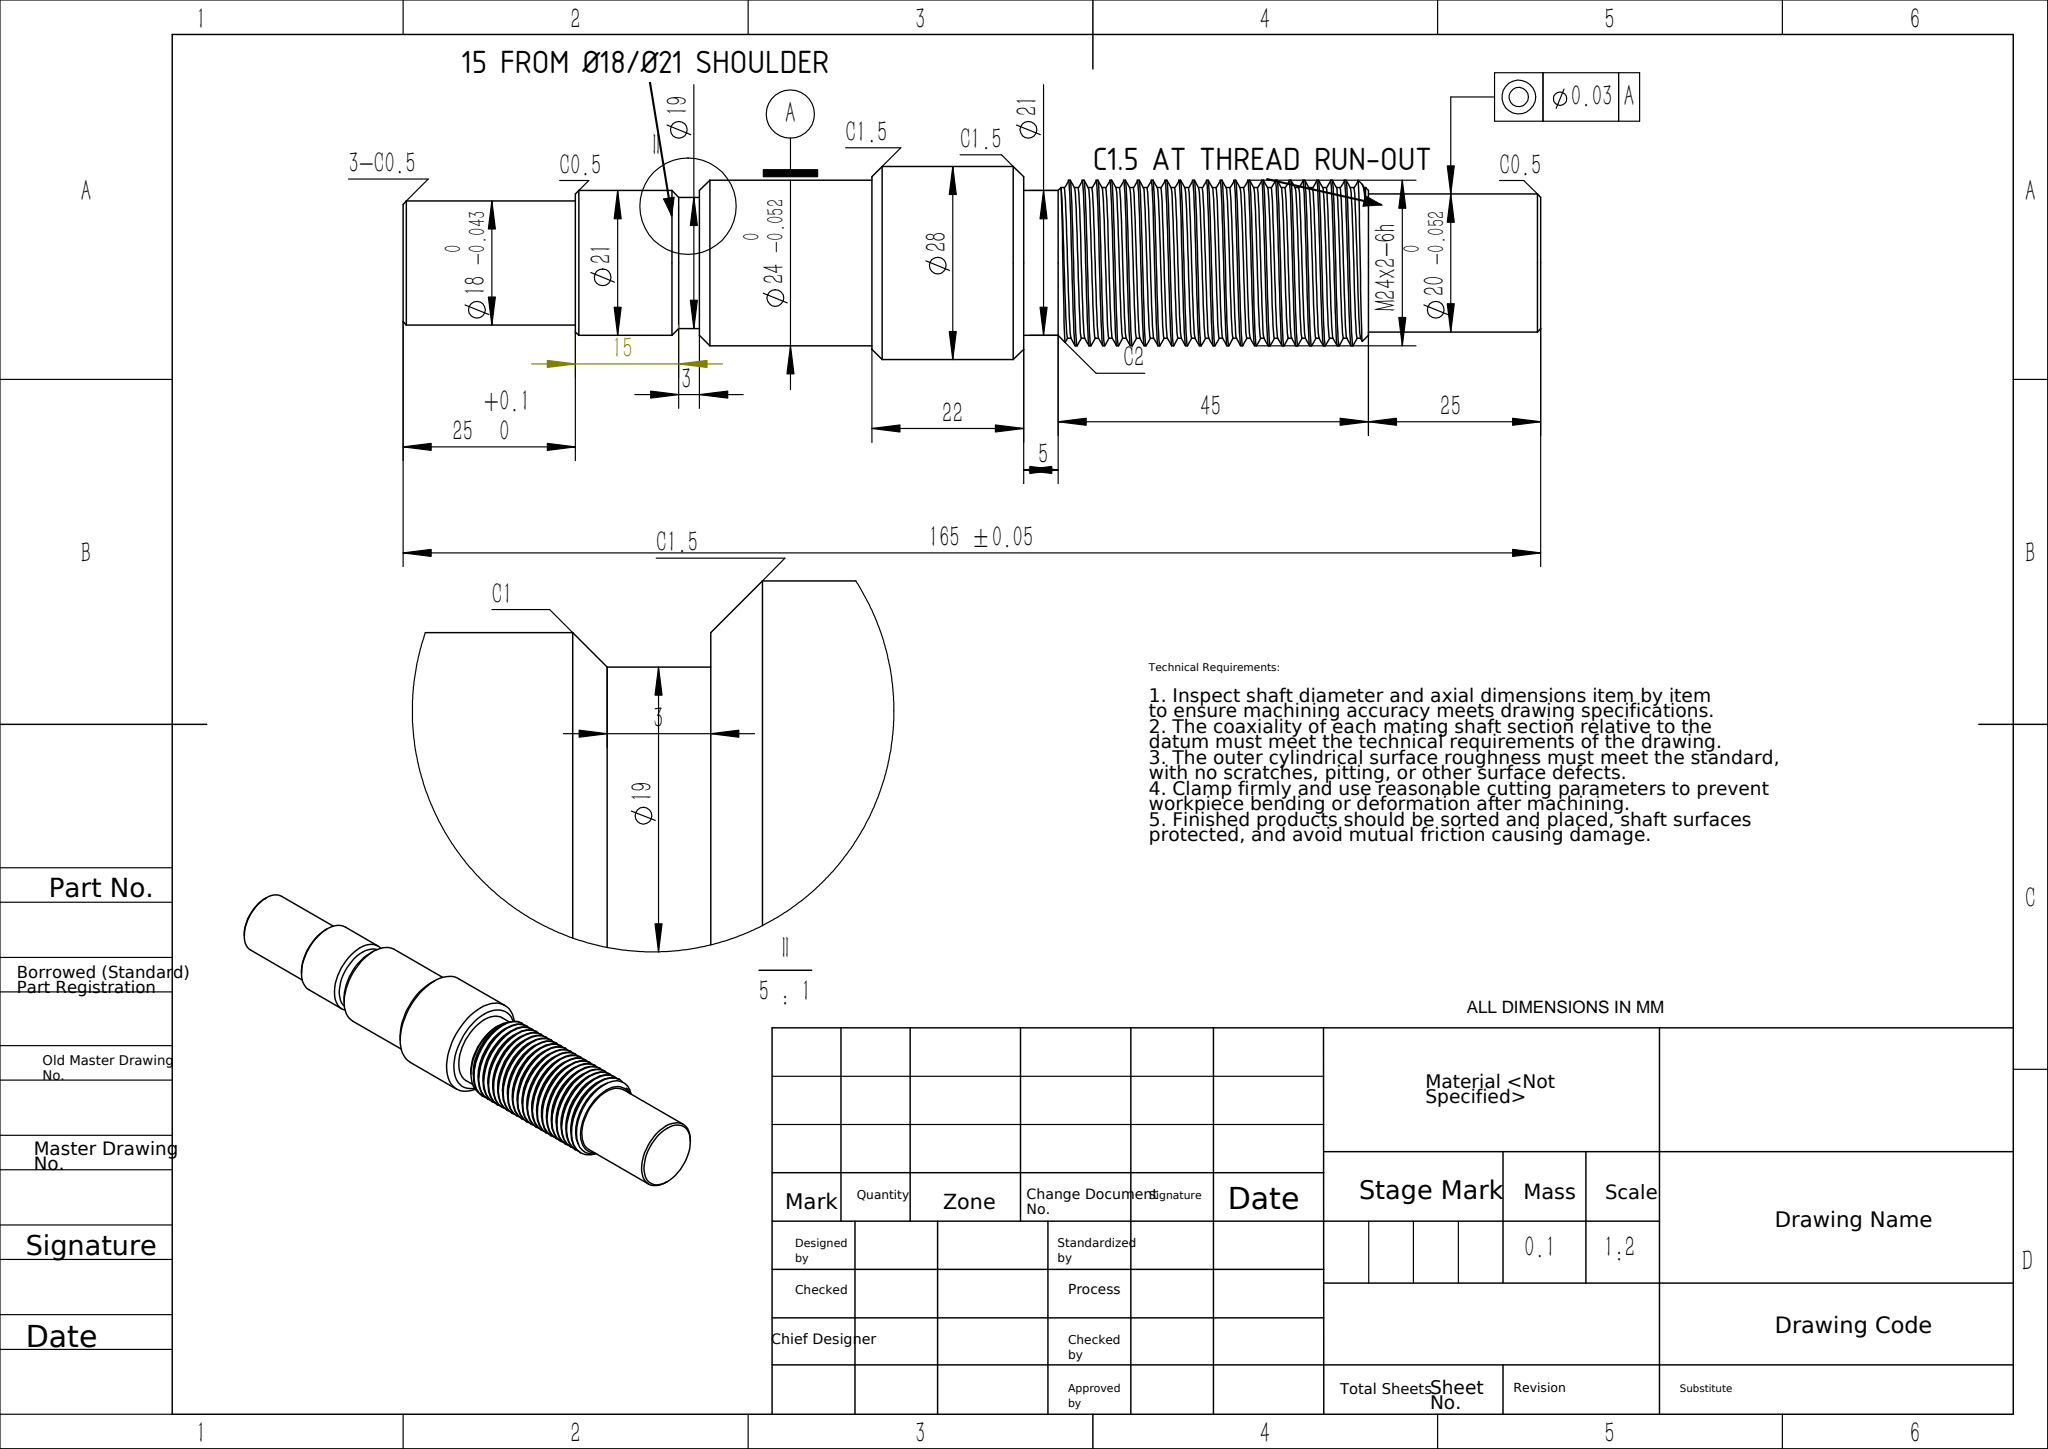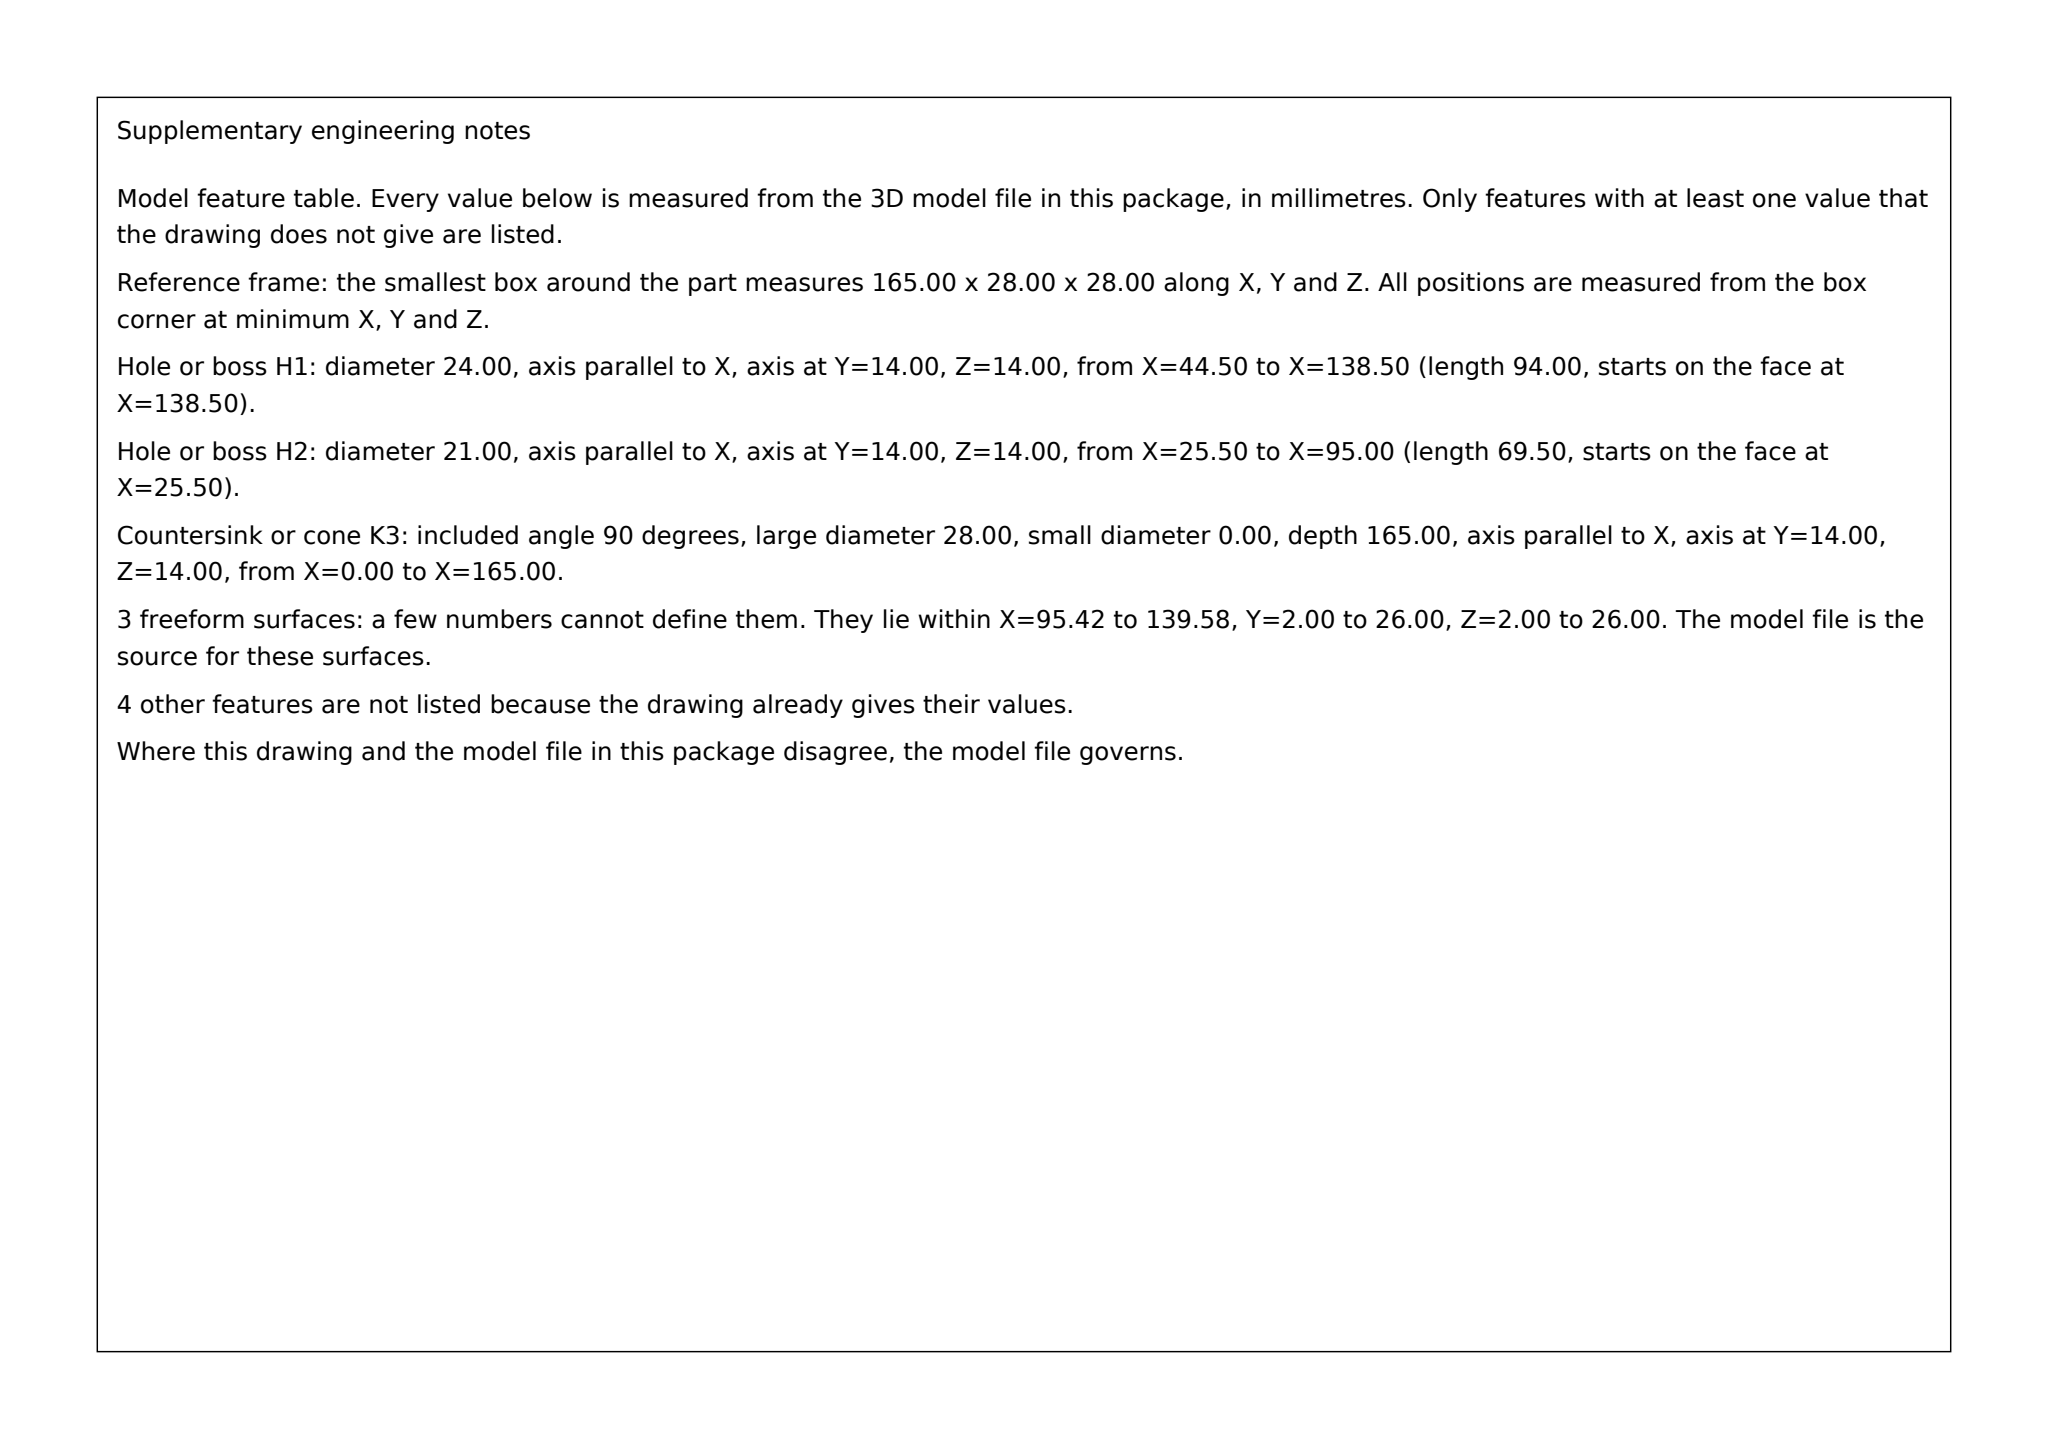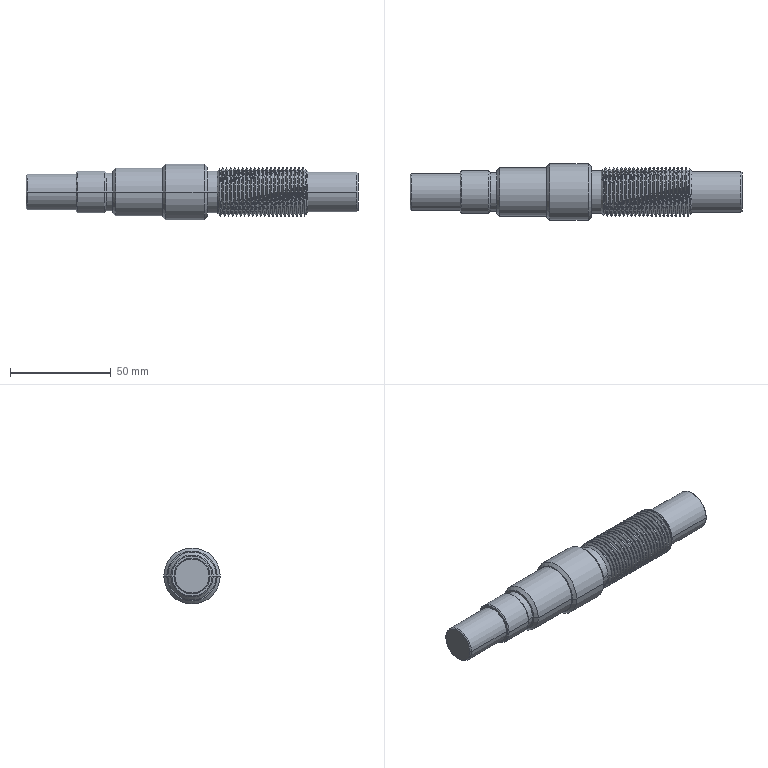Part | SolidWorks | mm | 1 solid | 85 faces | box 165 x 28 x 28 mm | volume 64827 mm3 | cylinder 57 | cone 18 | plane 7 | spline 3 | commonest cylinder face diameters 24 x45 21 x4 20 x2 28 x2 19 x2 18 x2
Drawing notes:
C1.5 AT THREAD RUN-OUT, M24X2 TO Ø20, 140 FROM LH END | from the solid: cone 90deg ref dia 21 at x=138.5-140, size 1.5; Ø20 shaft from x=140
15 = Ø18/Ø21 SHOULDER TO LH EDGE OF Ø19 GROOVE (3 WIDE) | from the solid: plane x=25 (Ø18/Ø21 shoulder) to Ø19 groove from x=40 to 43 => 15, groove 3